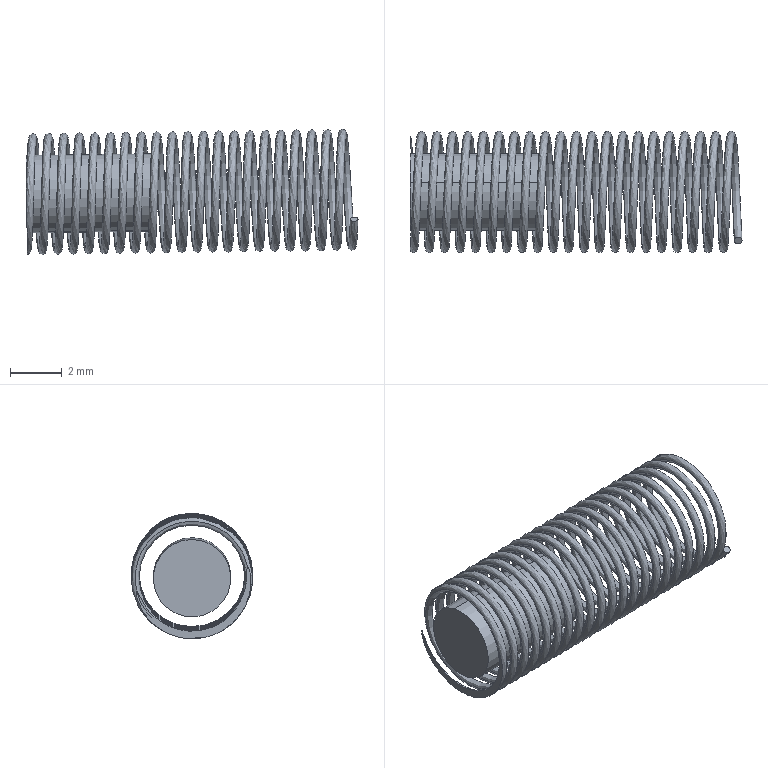Component | SolidWorks | PurchasedPart_5mmSmallSpring-1 | 2 solids | 8 faces | volume 56 mm3 | plane 4 | cylinder 2 | spline 2 | commonest cylinder face diameters 3 x2